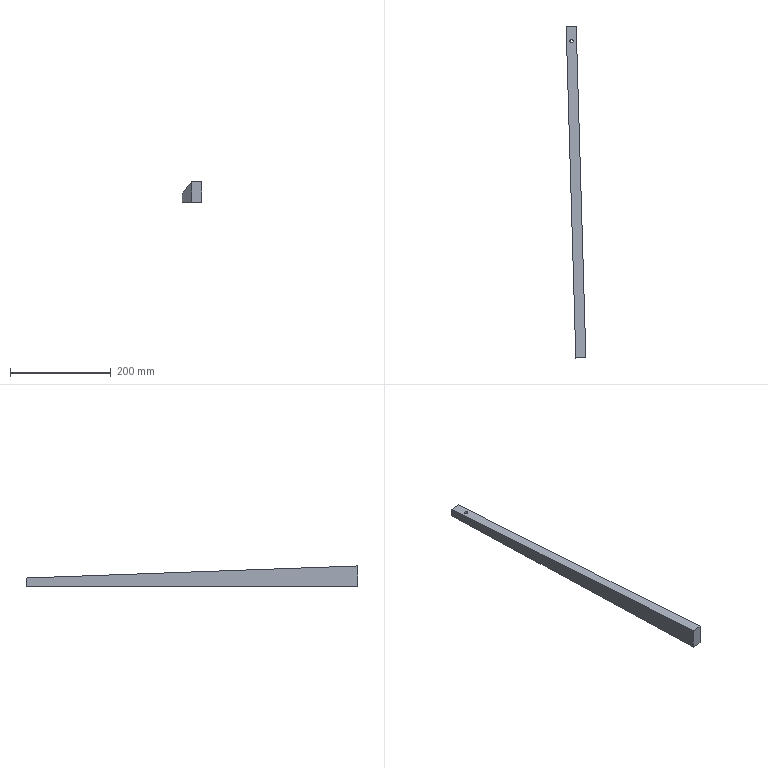Component | SolidWorks | Stiffener-1 | 1 solid | 20 faces | box 39.25 x 660.3 x 40 mm | volume 366753 mm3 | cylinder 8 | cone 6 | plane 6 | commonest cylinder face diameters 6.8 x8 | material 6063
build123d program:
from build123d import *

# Parameters (mm, degrees)
SKETCH1_W           = 660
SKETCH1_H           = 40
BOSS_EXTRUDE1_DEPTH = 10
CUT_EXTRUDE1_DEPTH  = 332.21
LPATTERN1_COUNT     = 4
LPATTERN1_PITCH     = 200


with BuildPart() as part:
    # Sketch1 → Boss-Extrude1 (new, symmetric)
    with BuildSketch(Plane.XY):
        Rectangle(SKETCH1_W, SKETCH1_H)
    extrude(amount=BOSS_EXTRUDE1_DEPTH, both=True)

    # Sketch2 → Cut-Extrude1 (cut, through all)
    with BuildSketch(Plane.XY.offset(10)):
        Polygon((-330, 20), (330, -4), (330, 20), align=None)
    extrude(amount=-CUT_EXTRUDE1_DEPTH, mode=Mode.SUBTRACT)

    # Sketch4 → M8 Tapped Hole1 (revolve, cut)
    with BuildSketch(Plane(origin=(-300, -20, 0), x_dir=(0, 0, -1), z_dir=(1, 0, 0))):
        Polygon((0, 0), (0, 21.793), (3.4, 19.75), (3.4, 0), align=None)
    m8_tapped_hole1 = revolve(axis=Axis((-300, -26.35, 0), (0, 1, 0)), mode=Mode.SUBTRACT)

    # LPattern1: M8 Tapped Hole1 ×4
    with Locations(*[(i * LPATTERN1_PITCH, 0, 0) for i in range(1, LPATTERN1_COUNT)]):
        add(m8_tapped_hole1, mode=Mode.SUBTRACT)


solid = part.part

# Placed as in the assembly
solid = solid.moved(Location((-293.326, 229.58, -1242.21), (-90, 88.328, -180)))
STEP:
#1=CARTESIAN_POINT('',(-11.759,20.848,-49.02));
#2=VERTEX_POINT('',#1);
#3=CARTESIAN_POINT('',(-12.027,20.841,-49.02));
#4=VERTEX_POINT('',#3);
#5=CARTESIAN_POINT('',(-11.759,20.848,-49.02));
#6=CARTESIAN_POINT('',(-11.751,20.581,-49.011));
#7=CARTESIAN_POINT('',(-12.019,20.573,-49.011));
#8=CARTESIAN_POINT('',(-12.027,20.841,-49.02));
#9=(BOUNDED_CURVE()B_SPLINE_CURVE(3,(#5,#6,#7,#8),.UNSPECIFIED.,.F.,.F.)B_SPLINE_CURVE_WITH_KNOTS((4,4),(1.571,4.712),.UNSPECIFIED.)CURVE()GEOMETRIC_REPRESENTATION_ITEM()RATIONAL_B_SPLINE_CURVE((1.,0.3333,0.3333,1.))REPRESENTATION_ITEM(''));
#10=EDGE_CURVE('',#2,#4,#9,.T.);
#11=ORIENTED_EDGE('',*,*,#10,.F.);
#12=CARTESIAN_POINT('',(-11.759,20.848,-49.693));
#13=VERTEX_POINT('',#12);
#14=CARTESIAN_POINT('',(-11.759,20.848,-49.693));
#15=DIRECTION('',(-0.,0.,-1.));
#16=VECTOR('',#15,39.37);
#17=LINE('',#14,#16);
#18=EDGE_CURVE('',#2,#13,#17,.T.);
#19=ORIENTED_EDGE('',*,*,#18,.T.);
#20=CARTESIAN_POINT('',(-12.027,20.841,-49.693));
#21=VERTEX_POINT('',#20);
#22=CARTESIAN_POINT('',(-11.893,20.845,-49.693));
#23=DIRECTION('',(-0.,0.,-1.));
#24=DIRECTION('',(-0.9996,-0.02918,0.));
#25=AXIS2_PLACEMENT_3D('',#22,#23,#24);
#26=CIRCLE('',#25,0.1339);
#27=EDGE_CURVE('',#13,#21,#26,.T.);
#28=ORIENTED_EDGE('',*,*,#27,.T.);
#29=CARTESIAN_POINT('',(-12.027,20.841,-49.693));
#30=DIRECTION('',(-0.,0.,-1.));
#31=VECTOR('',#30,39.37);
#32=LINE('',#29,#31);
#33=EDGE_CURVE('',#4,#21,#32,.T.);
#34=ORIENTED_EDGE('',*,*,#33,.F.);
#35=EDGE_LOOP('',(#11,#19,#28,#34));
#36=FACE_OUTER_BOUND('',#35,.T.);
#37=CARTESIAN_POINT('',(-11.893,20.845,-49.693));
#38=DIRECTION('',(-0.,0.,-1.));
#39=DIRECTION('',(-0.9996,-0.02918,0.));
#40=AXIS2_PLACEMENT_3D('',#37,#38,#39);
#41=CYLINDRICAL_SURFACE('',#40,0.1339);
#42=ADVANCED_FACE('',(#36),#41,.F.);
#43=CARTESIAN_POINT('',(-11.529,12.978,-48.916));
#44=VERTEX_POINT('',#43);
#45=CARTESIAN_POINT('',(-11.797,12.97,-48.916));
#46=VERTEX_POINT('',#45);
#47=CARTESIAN_POINT('',(-11.663,12.974,-48.916));
#48=DIRECTION('',(-0.,0.,-1.));
#49=DIRECTION('',(-0.9996,-0.02918,0.));
#50=AXIS2_PLACEMENT_3D('',#47,#48,#49);
#51=CIRCLE('',#50,0.1339);
#52=EDGE_CURVE('',#44,#46,#51,.T.);
#53=ORIENTED_EDGE('',*,*,#52,.F.);
#54=CARTESIAN_POINT('',(-11.529,12.978,-49.693));
#55=VERTEX_POINT('',#54);
#56=CARTESIAN_POINT('',(-11.529,12.978,-49.693));
#57=DIRECTION('',(-0.,0.,-1.));
#58=VECTOR('',#57,39.37);
#59=LINE('',#56,#58);
#60=EDGE_CURVE('',#44,#55,#59,.T.);
#61=ORIENTED_EDGE('',*,*,#60,.T.);
#62=CARTESIAN_POINT('',(-11.797,12.97,-49.693));
#63=VERTEX_POINT('',#62);
#64=CARTESIAN_POINT('',(-11.663,12.974,-49.693));
#65=DIRECTION('',(-0.,0.,-1.));
#66=DIRECTION('',(-0.9996,-0.02918,0.));
#67=AXIS2_PLACEMENT_3D('',#64,#65,#66);
#68=CIRCLE('',#67,0.1339);
#69=EDGE_CURVE('',#55,#63,#68,.T.);
#70=ORIENTED_EDGE('',*,*,#69,.T.);
#71=CARTESIAN_POINT('',(-11.797,12.97,-49.693));
#72=DIRECTION('',(-0.,0.,-1.));
#73=VECTOR('',#72,39.37);
#74=LINE('',#71,#73);
#75=EDGE_CURVE('',#46,#63,#74,.T.);
#76=ORIENTED_EDGE('',*,*,#75,.F.);
#77=EDGE_LOOP('',(#53,#61,#70,#76));
#78=FACE_OUTER_BOUND('',#77,.T.);
#79=CARTESIAN_POINT('',(-11.663,12.974,-49.693));
#80=DIRECTION('',(-0.,0.,-1.));
#81=DIRECTION('',(-0.9996,-0.02918,0.));
#82=AXIS2_PLACEMENT_3D('',#79,#80,#81);
#83=CYLINDRICAL_SURFACE('',#82,0.1339);
#84=ADVANCED_FACE('',(#78),#83,.F.);
#85=CARTESIAN_POINT('',(-11.663,12.974,-48.835));
#86=VERTEX_POINT('',#85);
#87=CARTESIAN_POINT('',(-11.797,12.97,-48.916));
#88=DIRECTION('',(-0.8568,-0.02501,-0.515));
#89=VECTOR('',#88,39.37);
#90=LINE('',#87,#89);
#91=EDGE_CURVE('',#86,#46,#90,.T.);
#92=ORIENTED_EDGE('',*,*,#91,.F.);
#93=CARTESIAN_POINT('',(-11.529,12.978,-48.916));
#94=DIRECTION('',(0.8568,0.02501,-0.515));
#95=VECTOR('',#94,39.37);
#96=LINE('',#93,#95);
#97=EDGE_CURVE('',#86,#44,#96,.T.);
#98=ORIENTED_EDGE('',*,*,#97,.T.);
#99=ORIENTED_EDGE('',*,*,#52,.T.);
#100=EDGE_LOOP('',(#92,#98,#99));
#101=FACE_OUTER_BOUND('',#100,.T.);
#102=CARTESIAN_POINT('',(-11.663,12.974,-48.916));
#103=DIRECTION('',(-0.,0.,-1.));
#104=DIRECTION('',(-0.9996,-0.02918,0.));
#105=AXIS2_PLACEMENT_3D('',#102,#103,#104);
#106=CONICAL_SURFACE('',#105,0.1339,1.03);
#107=ADVANCED_FACE('',(#101),#106,.F.);
#108=CARTESIAN_POINT('',(-11.3,5.107,-48.916));
#109=VERTEX_POINT('',#108);
#110=CARTESIAN_POINT('',(-11.567,5.099,-48.916));
#111=VERTEX_POINT('',#110);
#112=CARTESIAN_POINT('',(-11.433,5.103,-48.916));
#113=DIRECTION('',(-0.,0.,-1.));
#114=DIRECTION('',(-0.9996,-0.02918,0.));
#115=AXIS2_PLACEMENT_3D('',#112,#113,#114);
#116=CIRCLE('',#115,0.1339);
#117=EDGE_CURVE('',#109,#111,#116,.T.);
#118=ORIENTED_EDGE('',*,*,#117,.F.);
#119=CARTESIAN_POINT('',(-11.3,5.107,-49.693));
#120=VERTEX_POINT('',#119);
#121=CARTESIAN_POINT('',(-11.3,5.107,-49.693));
#122=DIRECTION('',(-0.,0.,-1.));
#123=VECTOR('',#122,39.37);
#124=LINE('',#121,#123);
#125=EDGE_CURVE('',#109,#120,#124,.T.);
#126=ORIENTED_EDGE('',*,*,#125,.T.);
#127=CARTESIAN_POINT('',(-11.567,5.099,-49.693));
#128=VERTEX_POINT('',#127);
#129=CARTESIAN_POINT('',(-11.433,5.103,-49.693));
#130=DIRECTION('',(-0.,0.,-1.));
#131=DIRECTION('',(-0.9996,-0.02918,0.));
#132=AXIS2_PLACEMENT_3D('',#129,#130,#131);
#133=CIRCLE('',#132,0.1339);
#134=EDGE_CURVE('',#120,#128,#133,.T.);
#135=ORIENTED_EDGE('',*,*,#134,.T.);
#136=CARTESIAN_POINT('',(-11.567,5.099,-49.693));
#137=DIRECTION('',(-0.,0.,-1.));
#138=VECTOR('',#137,39.37);
#139=LINE('',#136,#138);
#140=EDGE_CURVE('',#111,#128,#139,.T.);
#141=ORIENTED_EDGE('',*,*,#140,.F.);
#142=EDGE_LOOP('',(#118,#126,#135,#141));
#143=FACE_OUTER_BOUND('',#142,.T.);
#144=CARTESIAN_POINT('',(-11.433,5.103,-49.693));
#145=DIRECTION('',(-0.,0.,-1.));
#146=DIRECTION('',(-0.9996,-0.02918,0.));
#147=AXIS2_PLACEMENT_3D('',#144,#145,#146);
#148=CYLINDRICAL_SURFACE('',#147,0.1339);
#149=ADVANCED_FACE('',(#143),#148,.F.);
#150=CARTESIAN_POINT('',(-11.433,5.103,-48.835));
#151=VERTEX_POINT('',#150);
#152=CARTESIAN_POINT('',(-11.567,5.099,-48.916));
#153=DIRECTION('',(-0.8568,-0.02501,-0.515));
#154=VECTOR('',#153,39.37);
#155=LINE('',#152,#154);
#156=EDGE_CURVE('',#151,#111,#155,.T.);
#157=ORIENTED_EDGE('',*,*,#156,.F.);
#158=CARTESIAN_POINT('',(-11.3,5.107,-48.916));
#159=DIRECTION('',(0.8568,0.02501,-0.515));
#160=VECTOR('',#159,39.37);
#161=LINE('',#158,#160);
#162=EDGE_CURVE('',#151,#109,#161,.T.);
#163=ORIENTED_EDGE('',*,*,#162,.T.);
#164=ORIENTED_EDGE('',*,*,#117,.T.);
#165=EDGE_LOOP('',(#157,#163,#164));
#166=FACE_OUTER_BOUND('',#165,.T.);
#167=CARTESIAN_POINT('',(-11.433,5.103,-48.916));
#168=DIRECTION('',(-0.,0.,-1.));
#169=DIRECTION('',(-0.9996,-0.02918,0.));
#170=AXIS2_PLACEMENT_3D('',#167,#168,#169);
#171=CONICAL_SURFACE('',#170,0.1339,1.03);
#172=ADVANCED_FACE('',(#166),#171,.F.);
#173=CARTESIAN_POINT('',(-11.07,-2.764,-48.916));
#174=VERTEX_POINT('',#173);
#175=CARTESIAN_POINT('',(-11.337,-2.771,-48.916));
#176=VERTEX_POINT('',#175);
#177=CARTESIAN_POINT('',(-11.204,-2.767,-48.916));
#178=DIRECTION('',(-0.,0.,-1.));
#179=DIRECTION('',(-0.9996,-0.02918,0.));
#180=AXIS2_PLACEMENT_3D('',#177,#178,#179);
#181=CIRCLE('',#180,0.1339);
#182=EDGE_CURVE('',#174,#176,#181,.T.);
#183=ORIENTED_EDGE('',*,*,#182,.F.);
#184=CARTESIAN_POINT('',(-11.07,-2.764,-49.693));
#185=VERTEX_POINT('',#184);
#186=CARTESIAN_POINT('',(-11.07,-2.764,-49.693));
#187=DIRECTION('',(-0.,0.,-1.));
#188=VECTOR('',#187,39.37);
#189=LINE('',#186,#188);
#190=EDGE_CURVE('',#174,#185,#189,.T.);
#191=ORIENTED_EDGE('',*,*,#190,.T.);
#192=CARTESIAN_POINT('',(-11.337,-2.771,-49.693));
#193=VERTEX_POINT('',#192);
#194=CARTESIAN_POINT('',(-11.204,-2.767,-49.693));
#195=DIRECTION('',(-0.,0.,-1.));
#196=DIRECTION('',(-0.9996,-0.02918,0.));
#197=AXIS2_PLACEMENT_3D('',#194,#195,#196);
#198=CIRCLE('',#197,0.1339);
#199=EDGE_CURVE('',#185,#193,#198,.T.);
#200=ORIENTED_EDGE('',*,*,#199,.T.);
#201=CARTESIAN_POINT('',(-11.337,-2.771,-49.693));
#202=DIRECTION('',(-0.,0.,-1.));
#203=VECTOR('',#202,39.37);
#204=LINE('',#201,#203);
#205=EDGE_CURVE('',#176,#193,#204,.T.);
#206=ORIENTED_EDGE('',*,*,#205,.F.);
#207=EDGE_LOOP('',(#183,#191,#200,#206));
#208=FACE_OUTER_BOUND('',#207,.T.);
#209=CARTESIAN_POINT('',(-11.204,-2.767,-49.693));
#210=DIRECTION('',(-0.,0.,-1.));
#211=DIRECTION('',(-0.9996,-0.02918,0.));
#212=AXIS2_PLACEMENT_3D('',#209,#210,#211);
#213=CYLINDRICAL_SURFACE('',#212,0.1339);
#214=ADVANCED_FACE('',(#208),#213,.F.);
#215=CARTESIAN_POINT('',(-11.204,-2.767,-48.835));
#216=VERTEX_POINT('',#215);
#217=CARTESIAN_POINT('',(-11.337,-2.771,-48.916));
#218=DIRECTION('',(-0.8568,-0.02501,-0.515));
#219=VECTOR('',#218,39.37);
#220=LINE('',#217,#219);
#221=EDGE_CURVE('',#216,#176,#220,.T.);
#222=ORIENTED_EDGE('',*,*,#221,.F.);
#223=CARTESIAN_POINT('',(-11.07,-2.764,-48.916));
#224=DIRECTION('',(0.8568,0.02501,-0.515));
#225=VECTOR('',#224,39.37);
#226=LINE('',#223,#225);
#227=EDGE_CURVE('',#216,#174,#226,.T.);
#228=ORIENTED_EDGE('',*,*,#227,.T.);
#229=ORIENTED_EDGE('',*,*,#182,.T.);
#230=EDGE_LOOP('',(#222,#228,#229));
#231=FACE_OUTER_BOUND('',#230,.T.);
#232=CARTESIAN_POINT('',(-11.204,-2.767,-48.916));
#233=DIRECTION('',(-0.,0.,-1.));
#234=DIRECTION('',(-0.9996,-0.02918,0.));
#235=AXIS2_PLACEMENT_3D('',#232,#233,#234);
#236=CONICAL_SURFACE('',#235,0.1339,1.03);
#237=ADVANCED_FACE('',(#231),#236,.F.);
#238=CARTESIAN_POINT('',(-12.321,22.014,-49.693));
#239=VERTEX_POINT('',#238);
#240=CARTESIAN_POINT('',(-12.321,22.014,-49.063));
#241=VERTEX_POINT('',#240);
#242=CARTESIAN_POINT('',(-12.321,22.014,-48.118));
#243=DIRECTION('',(0.,-0.,1.));
#244=VECTOR('',#243,39.37);
#245=LINE('',#242,#244);
#246=EDGE_CURVE('',#239,#241,#245,.T.);
#247=ORIENTED_EDGE('',*,*,#246,.T.);
#248=CARTESIAN_POINT('',(-11.534,22.037,-49.063));
#249=VERTEX_POINT('',#248);
#250=CARTESIAN_POINT('',(-12.321,22.014,-49.063));
#251=DIRECTION('',(0.9996,0.02918,-0.));
#252=VECTOR('',#251,39.37);
#253=LINE('',#250,#252);
#254=EDGE_CURVE('',#241,#249,#253,.T.);
#255=ORIENTED_EDGE('',*,*,#254,.T.);
#256=CARTESIAN_POINT('',(-11.534,22.037,-49.693));
#257=VERTEX_POINT('',#256);
#258=CARTESIAN_POINT('',(-11.534,22.037,-48.118));
#259=DIRECTION('',(0.,-0.,1.));
#260=VECTOR('',#259,39.37);
#261=LINE('',#258,#260);
#262=EDGE_CURVE('',#257,#249,#261,.T.);
#263=ORIENTED_EDGE('',*,*,#262,.F.);
#264=CARTESIAN_POINT('',(-11.534,22.037,-49.693));
#265=DIRECTION('',(-0.9996,-0.02918,0.));
#266=VECTOR('',#265,39.37);
#267=LINE('',#264,#266);
#268=EDGE_CURVE('',#257,#239,#267,.T.);
#269=ORIENTED_EDGE('',*,*,#268,.T.);
#270=EDGE_LOOP('',(#247,#255,#263,#269));
#271=FACE_OUTER_BOUND('',#270,.T.);
#272=CARTESIAN_POINT('',(-11.534,22.037,-48.118));
#273=DIRECTION('',(0.02918,-0.9996,-0.));
#274=DIRECTION('',(0.9996,0.02918,-0.));
#275=AXIS2_PLACEMENT_3D('',#272,#273,#274);
#276=PLANE('',#275);
#277=ADVANCED_FACE('',(#271),#276,.F.);
#278=CARTESIAN_POINT('',(-11.563,-3.959,-48.118));
#279=VERTEX_POINT('',#278);
#280=CARTESIAN_POINT('',(-11.563,-3.959,-49.693));
#281=VERTEX_POINT('',#280);
#282=CARTESIAN_POINT('',(-11.563,-3.959,-48.118));
#283=DIRECTION('',(-0.,0.,-1.));
#284=VECTOR('',#283,39.37);
#285=LINE('',#282,#284);
#286=EDGE_CURVE('',#279,#281,#285,.T.);
#287=ORIENTED_EDGE('',*,*,#286,.T.);
#288=CARTESIAN_POINT('',(-10.776,-3.937,-49.693));
#289=VERTEX_POINT('',#288);
#290=CARTESIAN_POINT('',(-10.776,-3.937,-49.693));
#291=DIRECTION('',(-0.9996,-0.02918,0.));
#292=VECTOR('',#291,39.37);
#293=LINE('',#290,#292);
#294=EDGE_CURVE('',#289,#281,#293,.T.);
#295=ORIENTED_EDGE('',*,*,#294,.F.);
#296=CARTESIAN_POINT('',(-10.776,-3.937,-48.118));
#297=VERTEX_POINT('',#296);
#298=CARTESIAN_POINT('',(-10.776,-3.937,-48.118));
#299=DIRECTION('',(-0.,0.,-1.));
#300=VECTOR('',#299,39.37);
#301=LINE('',#298,#300);
#302=EDGE_CURVE('',#297,#289,#301,.T.);
#303=ORIENTED_EDGE('',*,*,#302,.F.);
#304=CARTESIAN_POINT('',(-10.776,-3.937,-48.118));
#305=DIRECTION('',(-0.9996,-0.02918,0.));
#306=VECTOR('',#305,39.37);
#307=LINE('',#304,#306);
#308=EDGE_CURVE('',#297,#279,#307,.T.);
#309=ORIENTED_EDGE('',*,*,#308,.T.);
#310=EDGE_LOOP('',(#287,#295,#303,#309));
#311=FACE_OUTER_BOUND('',#310,.T.);
#312=CARTESIAN_POINT('',(-10.776,-3.937,-48.118));
#313=DIRECTION('',(-0.02918,0.9996,0.));
#314=DIRECTION('',(-0.9996,-0.02918,0.));
#315=AXIS2_PLACEMENT_3D('',#312,#313,#314);
#316=PLANE('',#315);
#317=ADVANCED_FACE('',(#311),#316,.F.);
#318=CARTESIAN_POINT('',(-11.893,20.845,-49.693));
#319=DIRECTION('',(-0.,0.,-1.));
#320=DIRECTION('',(-0.9996,-0.02918,0.));
#321=AXIS2_PLACEMENT_3D('',#318,#319,#320);
#322=CIRCLE('',#321,0.1339);
#323=EDGE_CURVE('',#21,#13,#322,.T.);
#324=ORIENTED_EDGE('',*,*,#323,.F.);
#325=ORIENTED_EDGE('',*,*,#27,.F.);
#326=EDGE_LOOP('',(#324,#325));
#327=FACE_BOUND('',#326,.T.);
#328=CARTESIAN_POINT('',(-11.663,12.974,-49.693));
#329=DIRECTION('',(-0.,0.,-1.));
#330=DIRECTION('',(-0.9996,-0.02918,0.));
#331=AXIS2_PLACEMENT_3D('',#328,#329,#330);
#332=CIRCLE('',#331,0.1339);
#333=EDGE_CURVE('',#63,#55,#332,.T.);
#334=ORIENTED_EDGE('',*,*,#333,.F.);
#335=ORIENTED_EDGE('',*,*,#69,.F.);
#336=EDGE_LOOP('',(#334,#335));
#337=FACE_BOUND('',#336,.T.);
#338=CARTESIAN_POINT('',(-11.433,5.103,-49.693));
#339=DIRECTION('',(-0.,0.,-1.));
#340=DIRECTION('',(-0.9996,-0.02918,0.));
#341=AXIS2_PLACEMENT_3D('',#338,#339,#340);
#342=CIRCLE('',#341,0.1339);
#343=EDGE_CURVE('',#128,#120,#342,.T.);
#344=ORIENTED_EDGE('',*,*,#343,.F.);
#345=ORIENTED_EDGE('',*,*,#134,.F.);
#346=EDGE_LOOP('',(#344,#345));
#347=FACE_BOUND('',#346,.T.);
#348=CARTESIAN_POINT('',(-11.204,-2.767,-49.693));
#349=DIRECTION('',(-0.,0.,-1.));
#350=DIRECTION('',(-0.9996,-0.02918,0.));
#351=AXIS2_PLACEMENT_3D('',#348,#349,#350);
#352=CIRCLE('',#351,0.1339);
#353=EDGE_CURVE('',#193,#185,#352,.T.);
#354=ORIENTED_EDGE('',*,*,#353,.F.);
#355=ORIENTED_EDGE('',*,*,#199,.F.);
#356=EDGE_LOOP('',(#354,#355));
#357=FACE_BOUND('',#356,.T.);
#358=CARTESIAN_POINT('',(-11.563,-3.959,-49.693));
#359=DIRECTION('',(-0.02918,0.9996,0.));
#360=VECTOR('',#359,39.37);
#361=LINE('',#358,#360);
#362=EDGE_CURVE('',#281,#239,#361,.T.);
#363=ORIENTED_EDGE('',*,*,#362,.T.);
#364=ORIENTED_EDGE('',*,*,#268,.F.);
#365=CARTESIAN_POINT('',(-10.776,-3.937,-49.693));
#366=DIRECTION('',(-0.02918,0.9996,0.));
#367=VECTOR('',#366,39.37);
#368=LINE('',#365,#367);
#369=EDGE_CURVE('',#289,#257,#368,.T.);
#370=ORIENTED_EDGE('',*,*,#369,.F.);
#371=ORIENTED_EDGE('',*,*,#294,.T.);
#372=EDGE_LOOP('',(#363,#364,#370,#371));
#373=FACE_OUTER_BOUND('',#372,.T.);
#374=CARTESIAN_POINT('',(-10.776,-3.937,-49.693));
#375=DIRECTION('',(0.,-0.,1.));
#376=DIRECTION('',(0.9996,0.02918,-0.));
#377=AXIS2_PLACEMENT_3D('',#374,#375,#376);
#378=PLANE('',#377);
#379=ADVANCED_FACE('',(#327,#337,#347,#357,#373),#378,.F.);
#380=CARTESIAN_POINT('',(-10.776,-3.937,-48.118));
#381=DIRECTION('',(-0.02916,0.9989,-0.03634));
#382=VECTOR('',#381,39.37);
#383=LINE('',#380,#382);
#384=EDGE_CURVE('',#297,#249,#383,.T.);
#385=ORIENTED_EDGE('',*,*,#384,.F.);
#386=ORIENTED_EDGE('',*,*,#302,.T.);
#387=ORIENTED_EDGE('',*,*,#369,.T.);
#388=ORIENTED_EDGE('',*,*,#262,.T.);
#389=EDGE_LOOP('',(#385,#386,#387,#388));
#390=FACE_OUTER_BOUND('',#389,.T.);
#391=CARTESIAN_POINT('',(-11.155,9.05,-48.906));
#392=DIRECTION('',(0.9996,0.02918,-0.));
#393=DIRECTION('',(-0.02918,0.9996,0.));
#394=AXIS2_PLACEMENT_3D('',#391,#392,#393);
#395=PLANE('',#394);
#396=ADVANCED_FACE('',(#390),#395,.T.);
#397=ORIENTED_EDGE('',*,*,#286,.F.);
#398=CARTESIAN_POINT('',(-11.563,-3.959,-48.118));
#399=DIRECTION('',(-0.02916,0.9989,-0.03634));
#400=VECTOR('',#399,39.37);
#401=LINE('',#398,#400);
#402=EDGE_CURVE('',#279,#241,#401,.T.);
#403=ORIENTED_EDGE('',*,*,#402,.T.);
#404=ORIENTED_EDGE('',*,*,#246,.F.);
#405=ORIENTED_EDGE('',*,*,#362,.F.);
#406=EDGE_LOOP('',(#397,#403,#404,#405));
#407=FACE_OUTER_BOUND('',#406,.T.);
#408=CARTESIAN_POINT('',(-11.942,9.027,-48.906));
#409=DIRECTION('',(0.9996,0.02918,-0.));
#410=DIRECTION('',(-0.02918,0.9996,0.));
#411=AXIS2_PLACEMENT_3D('',#408,#409,#410);
#412=PLANE('',#411);
#413=ADVANCED_FACE('',(#407),#412,.F.);
#414=CARTESIAN_POINT('',(-12.027,20.841,-49.02));
#415=CARTESIAN_POINT('',(-12.035,21.108,-49.03));
#416=CARTESIAN_POINT('',(-11.767,21.116,-49.03));
#417=CARTESIAN_POINT('',(-11.759,20.848,-49.02));
#418=(BOUNDED_CURVE()B_SPLINE_CURVE(3,(#414,#415,#416,#417),.UNSPECIFIED.,.F.,.F.)B_SPLINE_CURVE_WITH_KNOTS((4,4),(4.712,7.854),.UNSPECIFIED.)CURVE()GEOMETRIC_REPRESENTATION_ITEM()RATIONAL_B_SPLINE_CURVE((1.,0.3333,0.3333,1.))REPRESENTATION_ITEM(''));
#419=EDGE_CURVE('',#4,#2,#418,.T.);
#420=ORIENTED_EDGE('',*,*,#419,.T.);
#421=ORIENTED_EDGE('',*,*,#10,.T.);
#422=EDGE_LOOP('',(#420,#421));
#423=FACE_BOUND('',#422,.T.);
#424=ORIENTED_EDGE('',*,*,#384,.T.);
#425=ORIENTED_EDGE('',*,*,#254,.F.);
#426=ORIENTED_EDGE('',*,*,#402,.F.);
#427=ORIENTED_EDGE('',*,*,#308,.F.);
#428=EDGE_LOOP('',(#424,#425,#426,#427));
#429=FACE_OUTER_BOUND('',#428,.T.);
#430=CARTESIAN_POINT('',(-11.563,-3.959,-48.118));
#431=DIRECTION('',(0.00106,-0.03632,-0.9993));
#432=DIRECTION('',(-0.02916,0.9989,-0.03634));
#433=AXIS2_PLACEMENT_3D('',#430,#431,#432);
#434=PLANE('',#433);
#435=ADVANCED_FACE('',(#423,#429),#434,.F.);
#436=ORIENTED_EDGE('',*,*,#227,.F.);
#437=ORIENTED_EDGE('',*,*,#221,.T.);
#438=CARTESIAN_POINT('',(-11.204,-2.767,-48.916));
#439=DIRECTION('',(-0.,0.,-1.));
#440=DIRECTION('',(-0.9996,-0.02918,0.));
#441=AXIS2_PLACEMENT_3D('',#438,#439,#440);
#442=CIRCLE('',#441,0.1339);
#443=EDGE_CURVE('',#176,#174,#442,.T.);
#444=ORIENTED_EDGE('',*,*,#443,.T.);
#445=EDGE_LOOP('',(#436,#437,#444));
#446=FACE_OUTER_BOUND('',#445,.T.);
#447=CARTESIAN_POINT('',(-11.204,-2.767,-48.916));
#448=DIRECTION('',(-0.,0.,-1.));
#449=DIRECTION('',(-0.9996,-0.02918,0.));
#450=AXIS2_PLACEMENT_3D('',#447,#448,#449);
#451=CONICAL_SURFACE('',#450,0.1339,1.03);
#452=ADVANCED_FACE('',(#446),#451,.F.);
#453=ORIENTED_EDGE('',*,*,#190,.F.);
#454=ORIENTED_EDGE('',*,*,#443,.F.);
#455=ORIENTED_EDGE('',*,*,#205,.T.);
#456=ORIENTED_EDGE('',*,*,#353,.T.);
#457=EDGE_LOOP('',(#453,#454,#455,#456));
#458=FACE_OUTER_BOUND('',#457,.T.);
#459=CARTESIAN_POINT('',(-11.204,-2.767,-49.693));
#460=DIRECTION('',(-0.,0.,-1.));
#461=DIRECTION('',(-0.9996,-0.02918,0.));
#462=AXIS2_PLACEMENT_3D('',#459,#460,#461);
#463=CYLINDRICAL_SURFACE('',#462,0.1339);
#464=ADVANCED_FACE('',(#458),#463,.F.);
#465=ORIENTED_EDGE('',*,*,#162,.F.);
#466=ORIENTED_EDGE('',*,*,#156,.T.);
#467=CARTESIAN_POINT('',(-11.433,5.103,-48.916));
#468=DIRECTION('',(-0.,0.,-1.));
#469=DIRECTION('',(-0.9996,-0.02918,0.));
#470=AXIS2_PLACEMENT_3D('',#467,#468,#469);
#471=CIRCLE('',#470,0.1339);
#472=EDGE_CURVE('',#111,#109,#471,.T.);
#473=ORIENTED_EDGE('',*,*,#472,.T.);
#474=EDGE_LOOP('',(#465,#466,#473));
#475=FACE_OUTER_BOUND('',#474,.T.);
#476=CARTESIAN_POINT('',(-11.433,5.103,-48.916));
#477=DIRECTION('',(-0.,0.,-1.));
#478=DIRECTION('',(-0.9996,-0.02918,0.));
#479=AXIS2_PLACEMENT_3D('',#476,#477,#478);
#480=CONICAL_SURFACE('',#479,0.1339,1.03);
#481=ADVANCED_FACE('',(#475),#480,.F.);
#482=ORIENTED_EDGE('',*,*,#125,.F.);
#483=ORIENTED_EDGE('',*,*,#472,.F.);
#484=ORIENTED_EDGE('',*,*,#140,.T.);
#485=ORIENTED_EDGE('',*,*,#343,.T.);
#486=EDGE_LOOP('',(#482,#483,#484,#485));
#487=FACE_OUTER_BOUND('',#486,.T.);
#488=CARTESIAN_POINT('',(-11.433,5.103,-49.693));
#489=DIRECTION('',(-0.,0.,-1.));
#490=DIRECTION('',(-0.9996,-0.02918,0.));
#491=AXIS2_PLACEMENT_3D('',#488,#489,#490);
#492=CYLINDRICAL_SURFACE('',#491,0.1339);
#493=ADVANCED_FACE('',(#487),#492,.F.);
#494=ORIENTED_EDGE('',*,*,#97,.F.);
#495=ORIENTED_EDGE('',*,*,#91,.T.);
#496=CARTESIAN_POINT('',(-11.663,12.974,-48.916));
#497=DIRECTION('',(-0.,0.,-1.));
#498=DIRECTION('',(-0.9996,-0.02918,0.));
#499=AXIS2_PLACEMENT_3D('',#496,#497,#498);
#500=CIRCLE('',#499,0.1339);
#501=EDGE_CURVE('',#46,#44,#500,.T.);
#502=ORIENTED_EDGE('',*,*,#501,.T.);
#503=EDGE_LOOP('',(#494,#495,#502));
#504=FACE_OUTER_BOUND('',#503,.T.);
#505=CARTESIAN_POINT('',(-11.663,12.974,-48.916));
#506=DIRECTION('',(-0.,0.,-1.));
#507=DIRECTION('',(-0.9996,-0.02918,0.));
#508=AXIS2_PLACEMENT_3D('',#505,#506,#507);
#509=CONICAL_SURFACE('',#508,0.1339,1.03);
#510=ADVANCED_FACE('',(#504),#509,.F.);
#511=ORIENTED_EDGE('',*,*,#60,.F.);
#512=ORIENTED_EDGE('',*,*,#501,.F.);
#513=ORIENTED_EDGE('',*,*,#75,.T.);
#514=ORIENTED_EDGE('',*,*,#333,.T.);
#515=EDGE_LOOP('',(#511,#512,#513,#514));
#516=FACE_OUTER_BOUND('',#515,.T.);
#517=CARTESIAN_POINT('',(-11.663,12.974,-49.693));
#518=DIRECTION('',(-0.,0.,-1.));
#519=DIRECTION('',(-0.9996,-0.02918,0.));
#520=AXIS2_PLACEMENT_3D('',#517,#518,#519);
#521=CYLINDRICAL_SURFACE('',#520,0.1339);
#522=ADVANCED_FACE('',(#516),#521,.F.);
#523=ORIENTED_EDGE('',*,*,#18,.F.);
#524=ORIENTED_EDGE('',*,*,#419,.F.);
#525=ORIENTED_EDGE('',*,*,#33,.T.);
#526=ORIENTED_EDGE('',*,*,#323,.T.);
#527=EDGE_LOOP('',(#523,#524,#525,#526));
#528=FACE_OUTER_BOUND('',#527,.T.);
#529=CARTESIAN_POINT('',(-11.893,20.845,-49.693));
#530=DIRECTION('',(-0.,0.,-1.));
#531=DIRECTION('',(-0.9996,-0.02918,0.));
#532=AXIS2_PLACEMENT_3D('',#529,#530,#531);
#533=CYLINDRICAL_SURFACE('',#532,0.1339);
#534=ADVANCED_FACE('',(#528),#533,.F.);
#535=CLOSED_SHELL('',(#42,#84,#107,#149,#172,#214,#237,#277,#317,#379,#396,#413,#435,#452,#464,#481,#493,#510,#522,#534));
#536=MANIFOLD_SOLID_BREP('',#535);
#537=CARTESIAN_POINT('',(0.,0.,0.));
#538=DIRECTION('',(0.,0.,1.));
#539=DIRECTION('',(1.,0.,0.));
#540=AXIS2_PLACEMENT_3D('',#537,#538,#539);
#541=(LENGTH_UNIT()NAMED_UNIT(*)SI_UNIT($,.METRE.));
#542=LENGTH_MEASURE_WITH_UNIT(LENGTH_MEASURE(0.0254),#541);
#543=DIMENSIONAL_EXPONENTS(1.,0.,0.,0.,0.,0.,0.);
#544=(CONVERSION_BASED_UNIT('',#542)LENGTH_UNIT()NAMED_UNIT(#543));
#545=UNCERTAINTY_MEASURE_WITH_UNIT(LENGTH_MEASURE(0.00001),#544,'','');
#546=(NAMED_UNIT(*)PLANE_ANGLE_UNIT()SI_UNIT($,.RADIAN.));
#547=(NAMED_UNIT(*)SI_UNIT($,.STERADIAN.)SOLID_ANGLE_UNIT());
#548=(GEOMETRIC_REPRESENTATION_CONTEXT(3)GLOBAL_UNCERTAINTY_ASSIGNED_CONTEXT((#545))GLOBAL_UNIT_ASSIGNED_CONTEXT((#544,#546,#547))REPRESENTATION_CONTEXT('',''));
#549=ADVANCED_BREP_SHAPE_REPRESENTATION('',(#536,#540),#548);
#550=COLOUR_RGB('',0.7922,0.8196,0.9333);
#551=FILL_AREA_STYLE_COLOUR('',#550);
#552=FILL_AREA_STYLE('',(#551));
#553=SURFACE_STYLE_FILL_AREA(#552);
#554=SURFACE_SIDE_STYLE('',(#553));
#555=SURFACE_STYLE_USAGE(.BOTH.,#554);
#556=PRESENTATION_STYLE_ASSIGNMENT((#555));
#557=STYLED_ITEM('',(#556),#536);
#558=PRESENTATION_LAYER_ASSIGNMENT('','',(#557));
#559=(LENGTH_UNIT()NAMED_UNIT(*)SI_UNIT($,.METRE.));
#560=LENGTH_MEASURE_WITH_UNIT(LENGTH_MEASURE(0.0254),#559);
#561=DIMENSIONAL_EXPONENTS(1.,0.,0.,0.,0.,0.,0.);
#562=(CONVERSION_BASED_UNIT('',#560)LENGTH_UNIT()NAMED_UNIT(#561));
#563=UNCERTAINTY_MEASURE_WITH_UNIT(LENGTH_MEASURE(0.00001),#562,'','');
#564=(NAMED_UNIT(*)PLANE_ANGLE_UNIT()SI_UNIT($,.RADIAN.));
#565=(NAMED_UNIT(*)SI_UNIT($,.STERADIAN.)SOLID_ANGLE_UNIT());
#566=(GEOMETRIC_REPRESENTATION_CONTEXT(3)GLOBAL_UNCERTAINTY_ASSIGNED_CONTEXT((#563))GLOBAL_UNIT_ASSIGNED_CONTEXT((#562,#564,#565))REPRESENTATION_CONTEXT('',''));
#567=MECHANICAL_DESIGN_GEOMETRIC_PRESENTATION_REPRESENTATION('',(#557),#566);